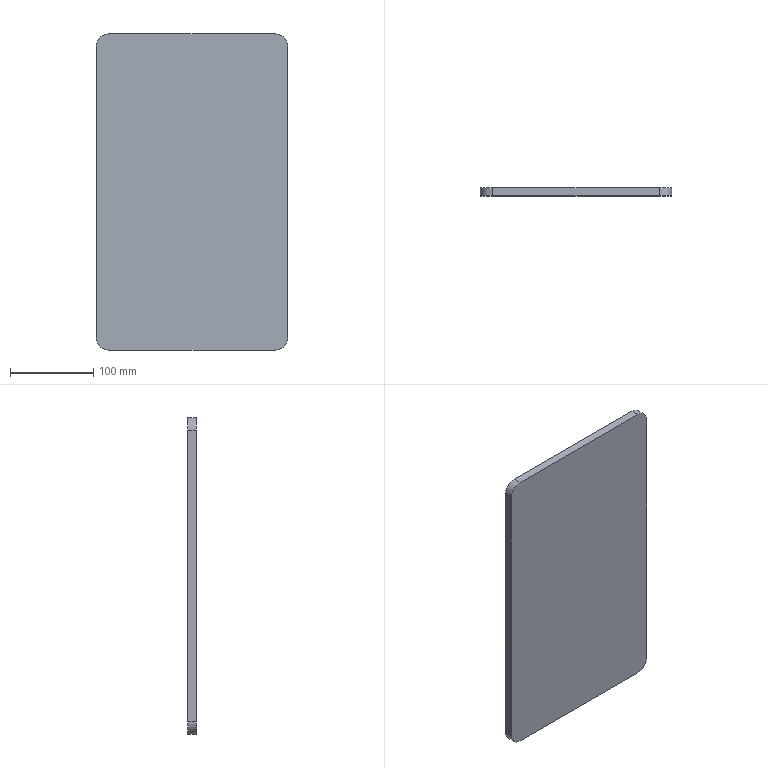Component | SolidWorks | Short-1_380X230X6-1 | 1 solid | 10 faces | box 230 x 10 x 380 mm | volume 872069 mm3 | plane 6 | cylinder 4 | commonest cylinder face diameters 30 x4 | material Plain Carbon Steel
STEP:
#1=COLOUR_RGB('',0.7922,0.8196,0.9333);
#2=FILL_AREA_STYLE_COLOUR('',#1);
#3=FILL_AREA_STYLE('',(#2));
#4=SURFACE_STYLE_FILL_AREA(#3);
#5=SURFACE_SIDE_STYLE('',(#4));
#6=SURFACE_STYLE_USAGE(.BOTH.,#5);
#7=PRESENTATION_STYLE_ASSIGNMENT((#6));
#8=CARTESIAN_POINT('',(-123.512,92.375,203.778));
#9=VERTEX_POINT('',#8);
#10=CARTESIAN_POINT('',(-122.921,92.375,203.188));
#11=VERTEX_POINT('',#10);
#12=CARTESIAN_POINT('',(-123.512,92.375,203.188));
#13=DIRECTION('',(0.,1.,-0.));
#14=DIRECTION('',(1.,0.,0.));
#15=AXIS2_PLACEMENT_3D('',#12,#13,#14);
#16=CIRCLE('',#15,0.5906);
#17=EDGE_CURVE('',#9,#11,#16,.T.);
#18=ORIENTED_EDGE('',*,*,#17,.F.);
#19=CARTESIAN_POINT('',(-123.512,91.981,203.778));
#20=VERTEX_POINT('',#19);
#21=CARTESIAN_POINT('',(-123.512,91.981,203.778));
#22=DIRECTION('',(0.,1.,-0.));
#23=VECTOR('',#22,39.37);
#24=LINE('',#21,#23);
#25=EDGE_CURVE('',#20,#9,#24,.T.);
#26=ORIENTED_EDGE('',*,*,#25,.F.);
#27=CARTESIAN_POINT('',(-122.921,91.981,203.188));
#28=VERTEX_POINT('',#27);
#29=CARTESIAN_POINT('',(-123.512,91.981,203.188));
#30=DIRECTION('',(0.,1.,-0.));
#31=DIRECTION('',(1.,0.,0.));
#32=AXIS2_PLACEMENT_3D('',#29,#30,#31);
#33=CIRCLE('',#32,0.5906);
#34=EDGE_CURVE('',#20,#28,#33,.T.);
#35=ORIENTED_EDGE('',*,*,#34,.T.);
#36=CARTESIAN_POINT('',(-122.921,91.981,203.188));
#37=DIRECTION('',(0.,1.,-0.));
#38=VECTOR('',#37,39.37);
#39=LINE('',#36,#38);
#40=EDGE_CURVE('',#28,#11,#39,.T.);
#41=ORIENTED_EDGE('',*,*,#40,.T.);
#42=EDGE_LOOP('',(#18,#26,#35,#41));
#43=FACE_OUTER_BOUND('',#42,.T.);
#44=CARTESIAN_POINT('',(-123.512,91.981,203.188));
#45=DIRECTION('',(0.,1.,-0.));
#46=DIRECTION('',(-1.,0.,0.));
#47=AXIS2_PLACEMENT_3D('',#44,#45,#46);
#48=CYLINDRICAL_SURFACE('',#47,0.5906);
#49=ADVANCED_FACE('',(#43),#48,.T.);
#50=CARTESIAN_POINT('',(-131.386,92.375,203.778));
#51=VERTEX_POINT('',#50);
#52=CARTESIAN_POINT('',(-123.512,92.375,203.778));
#53=DIRECTION('',(1.,-0.,-0.));
#54=VECTOR('',#53,39.37);
#55=LINE('',#52,#54);
#56=EDGE_CURVE('',#51,#9,#55,.T.);
#57=ORIENTED_EDGE('',*,*,#56,.F.);
#58=CARTESIAN_POINT('',(-131.386,91.981,203.778));
#59=VERTEX_POINT('',#58);
#60=CARTESIAN_POINT('',(-131.386,91.981,203.778));
#61=DIRECTION('',(0.,1.,-0.));
#62=VECTOR('',#61,39.37);
#63=LINE('',#60,#62);
#64=EDGE_CURVE('',#59,#51,#63,.T.);
#65=ORIENTED_EDGE('',*,*,#64,.F.);
#66=CARTESIAN_POINT('',(-123.512,91.981,203.778));
#67=DIRECTION('',(1.,-0.,-0.));
#68=VECTOR('',#67,39.37);
#69=LINE('',#66,#68);
#70=EDGE_CURVE('',#59,#20,#69,.T.);
#71=ORIENTED_EDGE('',*,*,#70,.T.);
#72=ORIENTED_EDGE('',*,*,#25,.T.);
#73=EDGE_LOOP('',(#57,#65,#71,#72));
#74=FACE_OUTER_BOUND('',#73,.T.);
#75=CARTESIAN_POINT('',(-123.512,91.981,203.778));
#76=DIRECTION('',(0.,0.,1.));
#77=DIRECTION('',(1.,-0.,-0.));
#78=AXIS2_PLACEMENT_3D('',#75,#76,#77);
#79=PLANE('',#78);
#80=ADVANCED_FACE('',(#74),#79,.T.);
#81=CARTESIAN_POINT('',(-131.976,92.375,203.188));
#82=VERTEX_POINT('',#81);
#83=CARTESIAN_POINT('',(-131.386,92.375,203.188));
#84=DIRECTION('',(0.,1.,-0.));
#85=DIRECTION('',(-1.,0.,0.));
#86=AXIS2_PLACEMENT_3D('',#83,#84,#85);
#87=CIRCLE('',#86,0.5906);
#88=EDGE_CURVE('',#82,#51,#87,.T.);
#89=ORIENTED_EDGE('',*,*,#88,.F.);
#90=CARTESIAN_POINT('',(-131.976,91.981,203.188));
#91=VERTEX_POINT('',#90);
#92=CARTESIAN_POINT('',(-131.976,91.981,203.188));
#93=DIRECTION('',(0.,1.,-0.));
#94=VECTOR('',#93,39.37);
#95=LINE('',#92,#94);
#96=EDGE_CURVE('',#91,#82,#95,.T.);
#97=ORIENTED_EDGE('',*,*,#96,.F.);
#98=CARTESIAN_POINT('',(-131.386,91.981,203.188));
#99=DIRECTION('',(0.,1.,-0.));
#100=DIRECTION('',(-1.,0.,0.));
#101=AXIS2_PLACEMENT_3D('',#98,#99,#100);
#102=CIRCLE('',#101,0.5906);
#103=EDGE_CURVE('',#91,#59,#102,.T.);
#104=ORIENTED_EDGE('',*,*,#103,.T.);
#105=ORIENTED_EDGE('',*,*,#64,.T.);
#106=EDGE_LOOP('',(#89,#97,#104,#105));
#107=FACE_OUTER_BOUND('',#106,.T.);
#108=CARTESIAN_POINT('',(-131.386,91.981,203.188));
#109=DIRECTION('',(0.,1.,-0.));
#110=DIRECTION('',(-1.,0.,0.));
#111=AXIS2_PLACEMENT_3D('',#108,#109,#110);
#112=CYLINDRICAL_SURFACE('',#111,0.5906);
#113=ADVANCED_FACE('',(#107),#112,.T.);
#114=CARTESIAN_POINT('',(-131.976,92.375,189.408));
#115=VERTEX_POINT('',#114);
#116=CARTESIAN_POINT('',(-131.976,92.375,189.408));
#117=DIRECTION('',(0.,0.,1.));
#118=VECTOR('',#117,39.37);
#119=LINE('',#116,#118);
#120=EDGE_CURVE('',#115,#82,#119,.T.);
#121=ORIENTED_EDGE('',*,*,#120,.F.);
#122=CARTESIAN_POINT('',(-131.976,91.981,189.408));
#123=VERTEX_POINT('',#122);
#124=CARTESIAN_POINT('',(-131.976,91.981,189.408));
#125=DIRECTION('',(0.,1.,-0.));
#126=VECTOR('',#125,39.37);
#127=LINE('',#124,#126);
#128=EDGE_CURVE('',#123,#115,#127,.T.);
#129=ORIENTED_EDGE('',*,*,#128,.F.);
#130=CARTESIAN_POINT('',(-131.976,91.981,189.408));
#131=DIRECTION('',(0.,0.,1.));
#132=VECTOR('',#131,39.37);
#133=LINE('',#130,#132);
#134=EDGE_CURVE('',#123,#91,#133,.T.);
#135=ORIENTED_EDGE('',*,*,#134,.T.);
#136=ORIENTED_EDGE('',*,*,#96,.T.);
#137=EDGE_LOOP('',(#121,#129,#135,#136));
#138=FACE_OUTER_BOUND('',#137,.T.);
#139=CARTESIAN_POINT('',(-131.976,91.981,189.408));
#140=DIRECTION('',(-1.,0.,0.));
#141=DIRECTION('',(0.,0.,1.));
#142=AXIS2_PLACEMENT_3D('',#139,#140,#141);
#143=PLANE('',#142);
#144=ADVANCED_FACE('',(#138),#143,.T.);
#145=CARTESIAN_POINT('',(-131.386,92.375,188.818));
#146=VERTEX_POINT('',#145);
#147=CARTESIAN_POINT('',(-131.386,92.375,189.408));
#148=DIRECTION('',(0.,1.,-0.));
#149=DIRECTION('',(-1.,0.,0.));
#150=AXIS2_PLACEMENT_3D('',#147,#148,#149);
#151=CIRCLE('',#150,0.5906);
#152=EDGE_CURVE('',#146,#115,#151,.T.);
#153=ORIENTED_EDGE('',*,*,#152,.F.);
#154=CARTESIAN_POINT('',(-131.386,91.981,188.818));
#155=VERTEX_POINT('',#154);
#156=CARTESIAN_POINT('',(-131.386,91.981,188.818));
#157=DIRECTION('',(0.,1.,-0.));
#158=VECTOR('',#157,39.37);
#159=LINE('',#156,#158);
#160=EDGE_CURVE('',#155,#146,#159,.T.);
#161=ORIENTED_EDGE('',*,*,#160,.F.);
#162=CARTESIAN_POINT('',(-131.386,91.981,189.408));
#163=DIRECTION('',(0.,1.,-0.));
#164=DIRECTION('',(-1.,0.,0.));
#165=AXIS2_PLACEMENT_3D('',#162,#163,#164);
#166=CIRCLE('',#165,0.5906);
#167=EDGE_CURVE('',#155,#123,#166,.T.);
#168=ORIENTED_EDGE('',*,*,#167,.T.);
#169=ORIENTED_EDGE('',*,*,#128,.T.);
#170=EDGE_LOOP('',(#153,#161,#168,#169));
#171=FACE_OUTER_BOUND('',#170,.T.);
#172=CARTESIAN_POINT('',(-131.386,91.981,189.408));
#173=DIRECTION('',(0.,1.,-0.));
#174=DIRECTION('',(-1.,0.,0.));
#175=AXIS2_PLACEMENT_3D('',#172,#173,#174);
#176=CYLINDRICAL_SURFACE('',#175,0.5906);
#177=ADVANCED_FACE('',(#171),#176,.T.);
#178=CARTESIAN_POINT('',(-123.512,92.375,188.818));
#179=VERTEX_POINT('',#178);
#180=CARTESIAN_POINT('',(-123.512,92.375,188.818));
#181=DIRECTION('',(-1.,0.,0.));
#182=VECTOR('',#181,39.37);
#183=LINE('',#180,#182);
#184=EDGE_CURVE('',#179,#146,#183,.T.);
#185=ORIENTED_EDGE('',*,*,#184,.F.);
#186=CARTESIAN_POINT('',(-123.512,91.981,188.818));
#187=VERTEX_POINT('',#186);
#188=CARTESIAN_POINT('',(-123.512,91.981,188.818));
#189=DIRECTION('',(0.,1.,-0.));
#190=VECTOR('',#189,39.37);
#191=LINE('',#188,#190);
#192=EDGE_CURVE('',#187,#179,#191,.T.);
#193=ORIENTED_EDGE('',*,*,#192,.F.);
#194=CARTESIAN_POINT('',(-123.512,91.981,188.818));
#195=DIRECTION('',(-1.,0.,0.));
#196=VECTOR('',#195,39.37);
#197=LINE('',#194,#196);
#198=EDGE_CURVE('',#187,#155,#197,.T.);
#199=ORIENTED_EDGE('',*,*,#198,.T.);
#200=ORIENTED_EDGE('',*,*,#160,.T.);
#201=EDGE_LOOP('',(#185,#193,#199,#200));
#202=FACE_OUTER_BOUND('',#201,.T.);
#203=CARTESIAN_POINT('',(-123.512,91.981,188.818));
#204=DIRECTION('',(-0.,-0.,-1.));
#205=DIRECTION('',(-1.,0.,0.));
#206=AXIS2_PLACEMENT_3D('',#203,#204,#205);
#207=PLANE('',#206);
#208=ADVANCED_FACE('',(#202),#207,.T.);
#209=CARTESIAN_POINT('',(-122.921,92.375,189.408));
#210=VERTEX_POINT('',#209);
#211=CARTESIAN_POINT('',(-123.512,92.375,189.408));
#212=DIRECTION('',(0.,1.,-0.));
#213=DIRECTION('',(-1.,0.,0.));
#214=AXIS2_PLACEMENT_3D('',#211,#212,#213);
#215=CIRCLE('',#214,0.5906);
#216=EDGE_CURVE('',#210,#179,#215,.T.);
#217=ORIENTED_EDGE('',*,*,#216,.F.);
#218=CARTESIAN_POINT('',(-122.921,91.981,189.408));
#219=VERTEX_POINT('',#218);
#220=CARTESIAN_POINT('',(-122.921,91.981,189.408));
#221=DIRECTION('',(0.,1.,-0.));
#222=VECTOR('',#221,39.37);
#223=LINE('',#220,#222);
#224=EDGE_CURVE('',#219,#210,#223,.T.);
#225=ORIENTED_EDGE('',*,*,#224,.F.);
#226=CARTESIAN_POINT('',(-123.512,91.981,189.408));
#227=DIRECTION('',(0.,1.,-0.));
#228=DIRECTION('',(-1.,0.,0.));
#229=AXIS2_PLACEMENT_3D('',#226,#227,#228);
#230=CIRCLE('',#229,0.5906);
#231=EDGE_CURVE('',#219,#187,#230,.T.);
#232=ORIENTED_EDGE('',*,*,#231,.T.);
#233=ORIENTED_EDGE('',*,*,#192,.T.);
#234=EDGE_LOOP('',(#217,#225,#232,#233));
#235=FACE_OUTER_BOUND('',#234,.T.);
#236=CARTESIAN_POINT('',(-123.512,91.981,189.408));
#237=DIRECTION('',(0.,1.,-0.));
#238=DIRECTION('',(-1.,0.,0.));
#239=AXIS2_PLACEMENT_3D('',#236,#237,#238);
#240=CYLINDRICAL_SURFACE('',#239,0.5906);
#241=ADVANCED_FACE('',(#235),#240,.T.);
#242=CARTESIAN_POINT('',(-122.921,92.375,189.408));
#243=DIRECTION('',(-0.,-0.,-1.));
#244=VECTOR('',#243,39.37);
#245=LINE('',#242,#244);
#246=EDGE_CURVE('',#11,#210,#245,.T.);
#247=ORIENTED_EDGE('',*,*,#246,.F.);
#248=ORIENTED_EDGE('',*,*,#40,.F.);
#249=CARTESIAN_POINT('',(-122.921,91.981,189.408));
#250=DIRECTION('',(-0.,-0.,-1.));
#251=VECTOR('',#250,39.37);
#252=LINE('',#249,#251);
#253=EDGE_CURVE('',#28,#219,#252,.T.);
#254=ORIENTED_EDGE('',*,*,#253,.T.);
#255=ORIENTED_EDGE('',*,*,#224,.T.);
#256=EDGE_LOOP('',(#247,#248,#254,#255));
#257=FACE_OUTER_BOUND('',#256,.T.);
#258=CARTESIAN_POINT('',(-122.921,91.981,189.408));
#259=DIRECTION('',(1.,-0.,-0.));
#260=DIRECTION('',(-0.,-0.,-1.));
#261=AXIS2_PLACEMENT_3D('',#258,#259,#260);
#262=PLANE('',#261);
#263=ADVANCED_FACE('',(#257),#262,.T.);
#264=ORIENTED_EDGE('',*,*,#34,.F.);
#265=ORIENTED_EDGE('',*,*,#70,.F.);
#266=ORIENTED_EDGE('',*,*,#103,.F.);
#267=ORIENTED_EDGE('',*,*,#134,.F.);
#268=ORIENTED_EDGE('',*,*,#167,.F.);
#269=ORIENTED_EDGE('',*,*,#198,.F.);
#270=ORIENTED_EDGE('',*,*,#231,.F.);
#271=ORIENTED_EDGE('',*,*,#253,.F.);
#272=EDGE_LOOP('',(#264,#265,#266,#267,#268,#269,#270,#271));
#273=FACE_OUTER_BOUND('',#272,.T.);
#274=CARTESIAN_POINT('',(-123.512,91.981,203.188));
#275=DIRECTION('',(-0.,-1.,0.));
#276=DIRECTION('',(1.,-0.,-0.));
#277=AXIS2_PLACEMENT_3D('',#274,#275,#276);
#278=PLANE('',#277);
#279=ADVANCED_FACE('',(#273),#278,.T.);
#280=ORIENTED_EDGE('',*,*,#17,.T.);
#281=ORIENTED_EDGE('',*,*,#246,.T.);
#282=ORIENTED_EDGE('',*,*,#216,.T.);
#283=ORIENTED_EDGE('',*,*,#184,.T.);
#284=ORIENTED_EDGE('',*,*,#152,.T.);
#285=ORIENTED_EDGE('',*,*,#120,.T.);
#286=ORIENTED_EDGE('',*,*,#88,.T.);
#287=ORIENTED_EDGE('',*,*,#56,.T.);
#288=EDGE_LOOP('',(#280,#281,#282,#283,#284,#285,#286,#287));
#289=FACE_OUTER_BOUND('',#288,.T.);
#290=CARTESIAN_POINT('',(-123.512,92.375,203.188));
#291=DIRECTION('',(-0.,-1.,0.));
#292=DIRECTION('',(1.,-0.,-0.));
#293=AXIS2_PLACEMENT_3D('',#290,#291,#292);
#294=PLANE('',#293);
#295=ADVANCED_FACE('',(#289),#294,.F.);
#296=CLOSED_SHELL('',(#49,#80,#113,#144,#177,#208,#241,#263,#279,#295));
#297=MANIFOLD_SOLID_BREP('',#296);
#298=STYLED_ITEM('',(#7),#297);
#299=(LENGTH_UNIT()NAMED_UNIT(*)SI_UNIT($,.METRE.));
#300=LENGTH_MEASURE_WITH_UNIT(LENGTH_MEASURE(0.0254),#299);
#301=DIMENSIONAL_EXPONENTS(1.,0.,0.,0.,0.,0.,0.);
#302=(CONVERSION_BASED_UNIT('',#300)LENGTH_UNIT()NAMED_UNIT(#301));
#303=UNCERTAINTY_MEASURE_WITH_UNIT(LENGTH_MEASURE(0.00001),#302,'','');
#304=(NAMED_UNIT(*)PLANE_ANGLE_UNIT()SI_UNIT($,.RADIAN.));
#305=(NAMED_UNIT(*)SI_UNIT($,.STERADIAN.)SOLID_ANGLE_UNIT());
#306=(GEOMETRIC_REPRESENTATION_CONTEXT(3)GLOBAL_UNCERTAINTY_ASSIGNED_CONTEXT((#303))GLOBAL_UNIT_ASSIGNED_CONTEXT((#302,#304,#305))REPRESENTATION_CONTEXT('',''));
#307=MECHANICAL_DESIGN_GEOMETRIC_PRESENTATION_REPRESENTATION('',(#298),#306);
#308=CARTESIAN_POINT('',(0.,0.,0.));
#309=DIRECTION('',(0.,0.,1.));
#310=DIRECTION('',(1.,0.,0.));
#311=AXIS2_PLACEMENT_3D('',#308,#309,#310);
#312=(LENGTH_UNIT()NAMED_UNIT(*)SI_UNIT($,.METRE.));
#313=LENGTH_MEASURE_WITH_UNIT(LENGTH_MEASURE(0.0254),#312);
#314=DIMENSIONAL_EXPONENTS(1.,0.,0.,0.,0.,0.,0.);
#315=(CONVERSION_BASED_UNIT('',#313)LENGTH_UNIT()NAMED_UNIT(#314));
#316=UNCERTAINTY_MEASURE_WITH_UNIT(LENGTH_MEASURE(0.00001),#315,'','');
#317=(NAMED_UNIT(*)PLANE_ANGLE_UNIT()SI_UNIT($,.RADIAN.));
#318=(NAMED_UNIT(*)SI_UNIT($,.STERADIAN.)SOLID_ANGLE_UNIT());
#319=(GEOMETRIC_REPRESENTATION_CONTEXT(3)GLOBAL_UNCERTAINTY_ASSIGNED_CONTEXT((#316))GLOBAL_UNIT_ASSIGNED_CONTEXT((#315,#317,#318))REPRESENTATION_CONTEXT('',''));
#320=ADVANCED_BREP_SHAPE_REPRESENTATION('',(#297,#311),#319);
#321=PRESENTATION_LAYER_ASSIGNMENT('','',(#298));